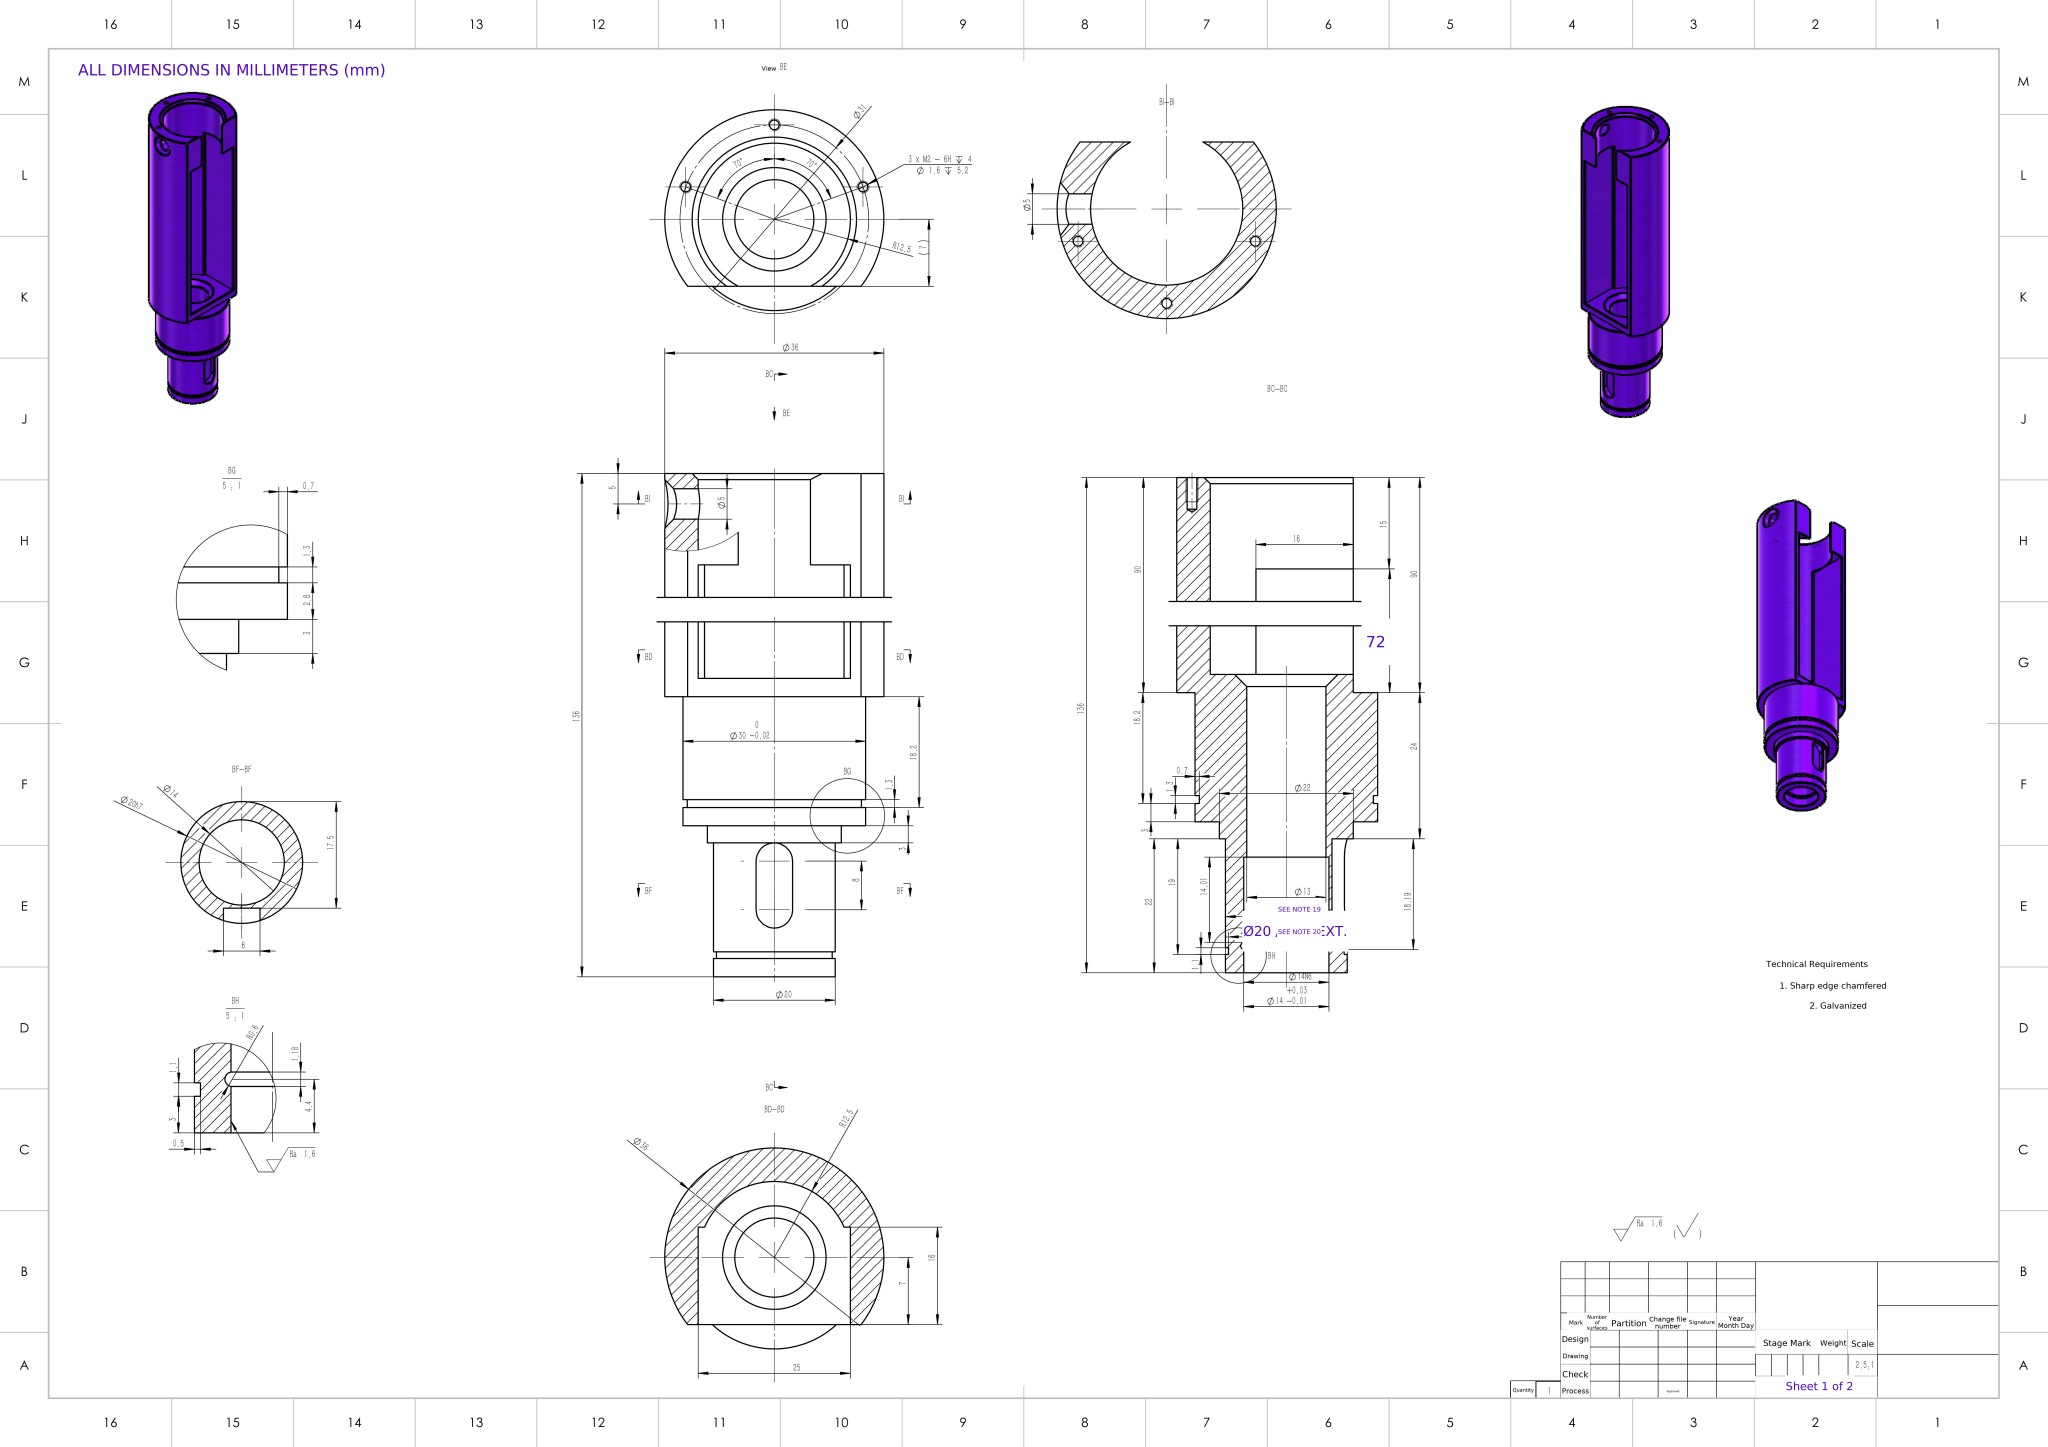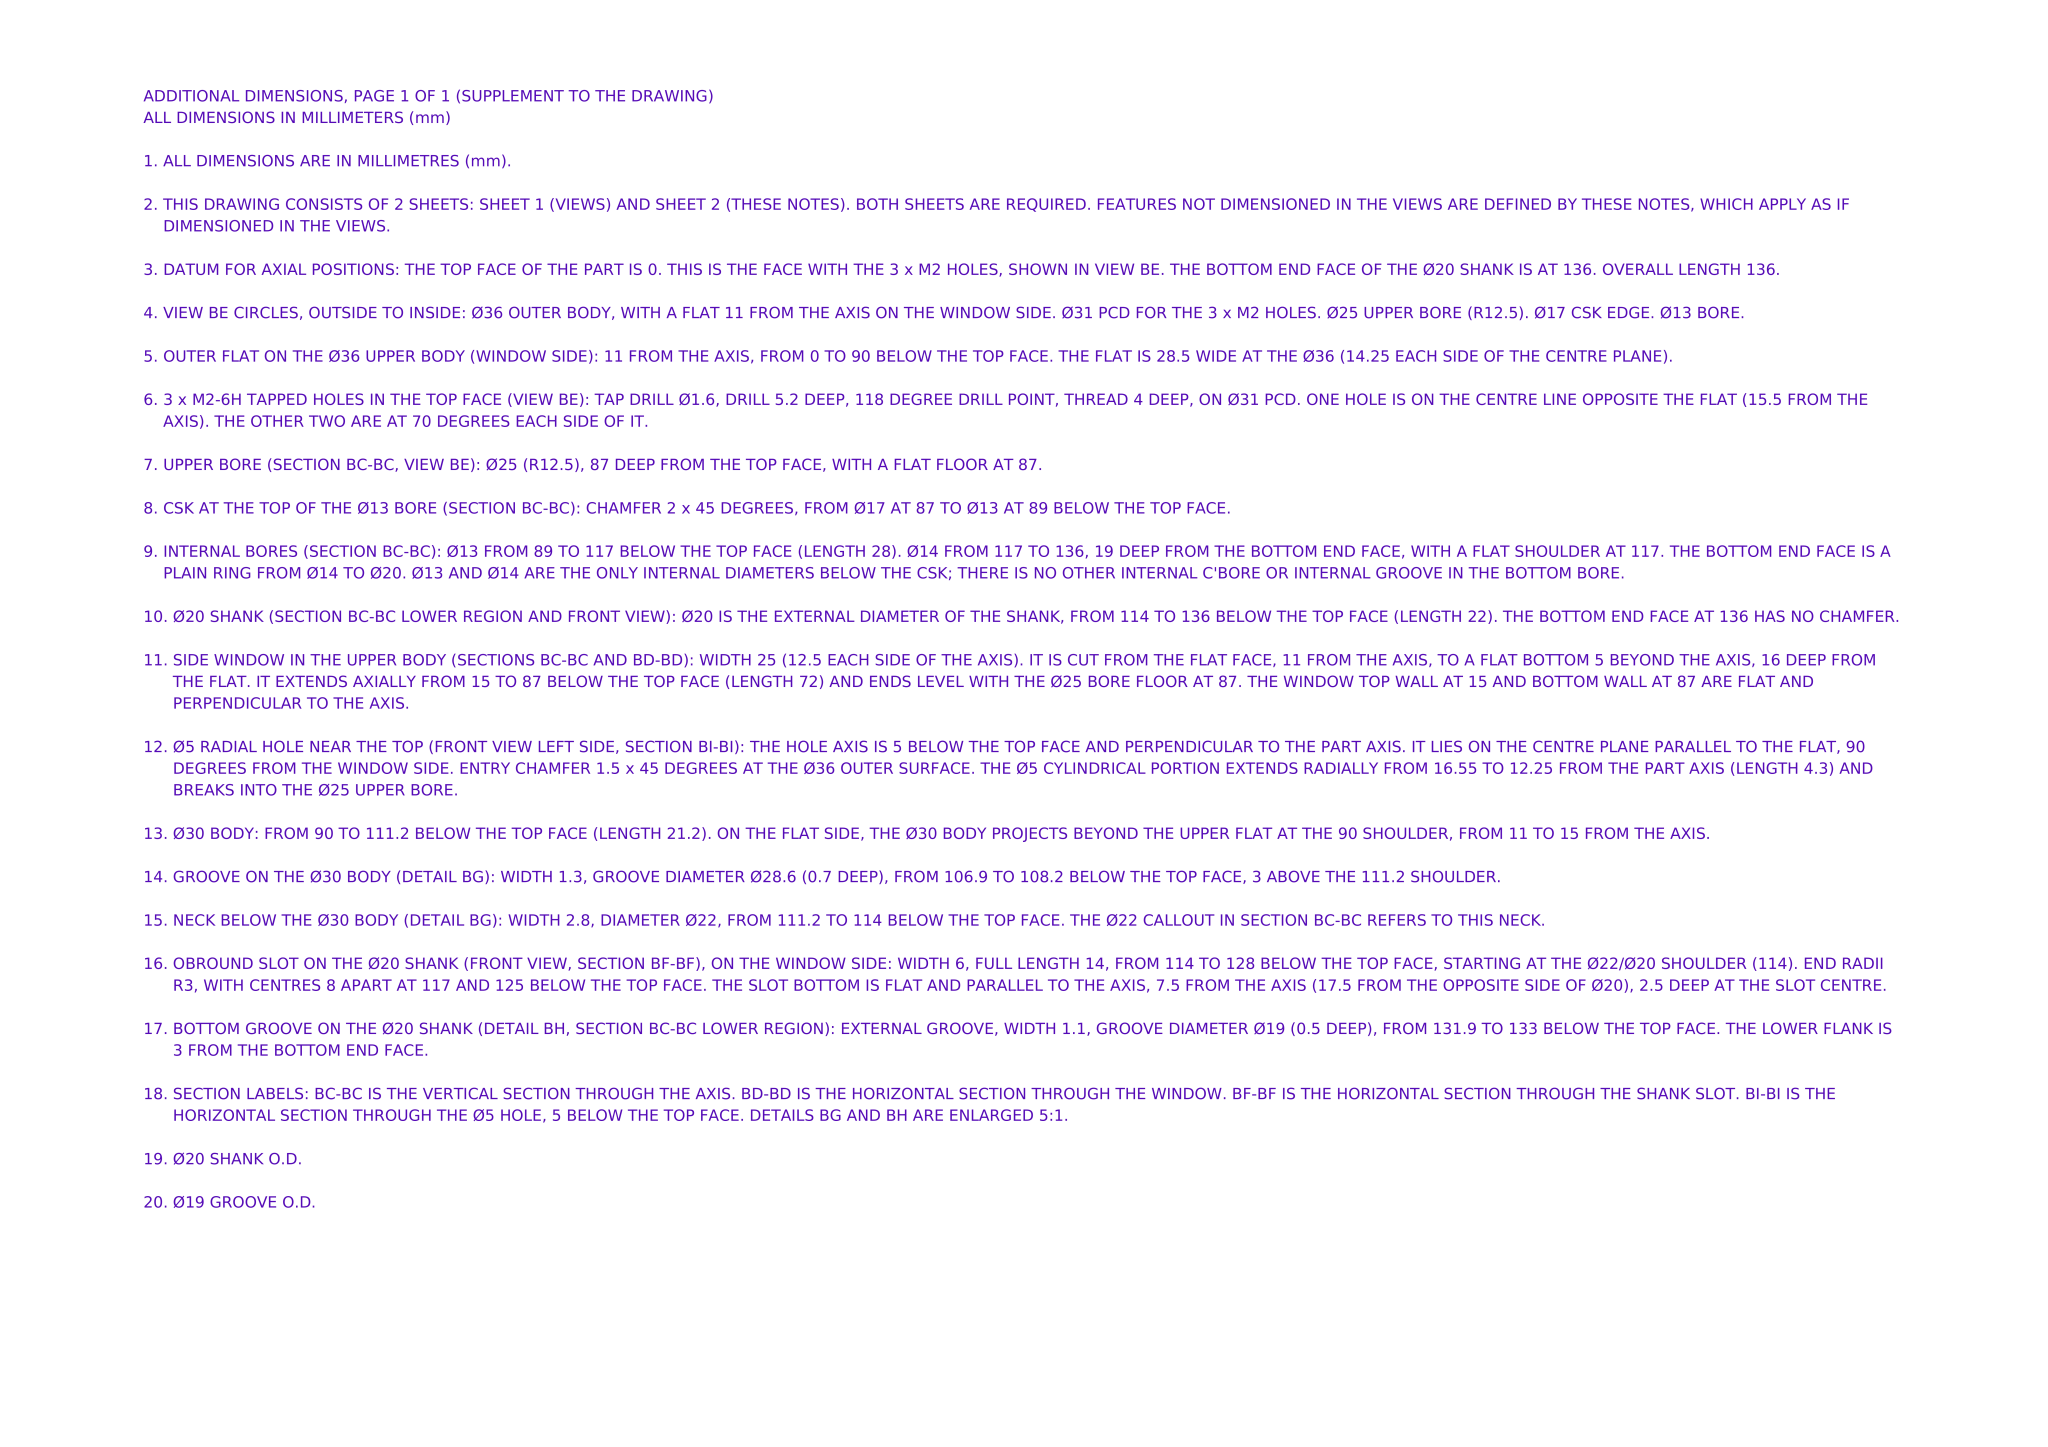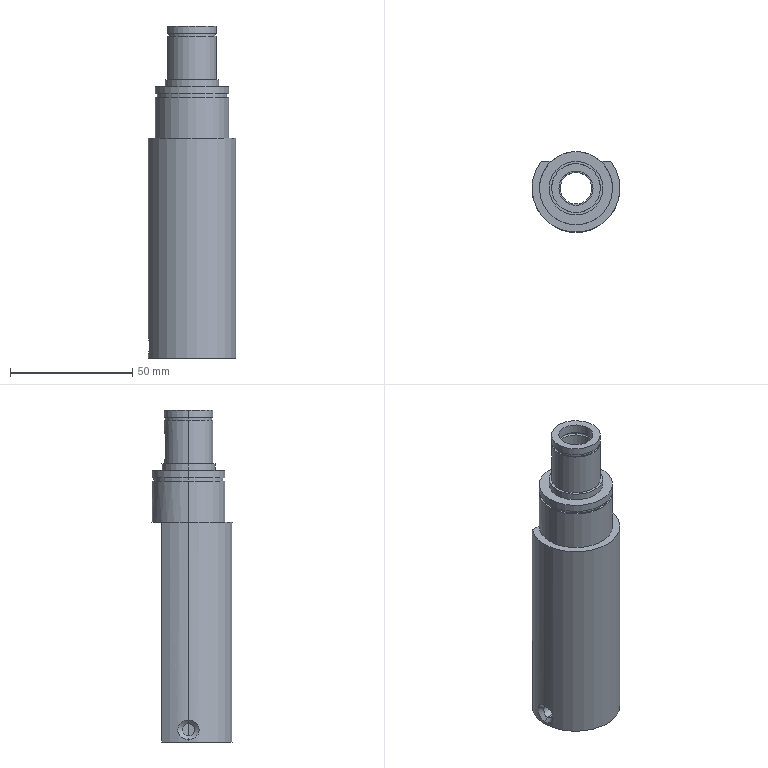Part | NX | mm | 1 solid | 78 faces | box 36 x 33 x 136 mm | volume 49627 mm3 | cylinder 37 | plane 24 | cone 11 | spline 6 | commonest cylinder face diameters 1.6 x6 30 x4 14 x4 20 x4 25 x3 36 x3 6 x3 5 x2